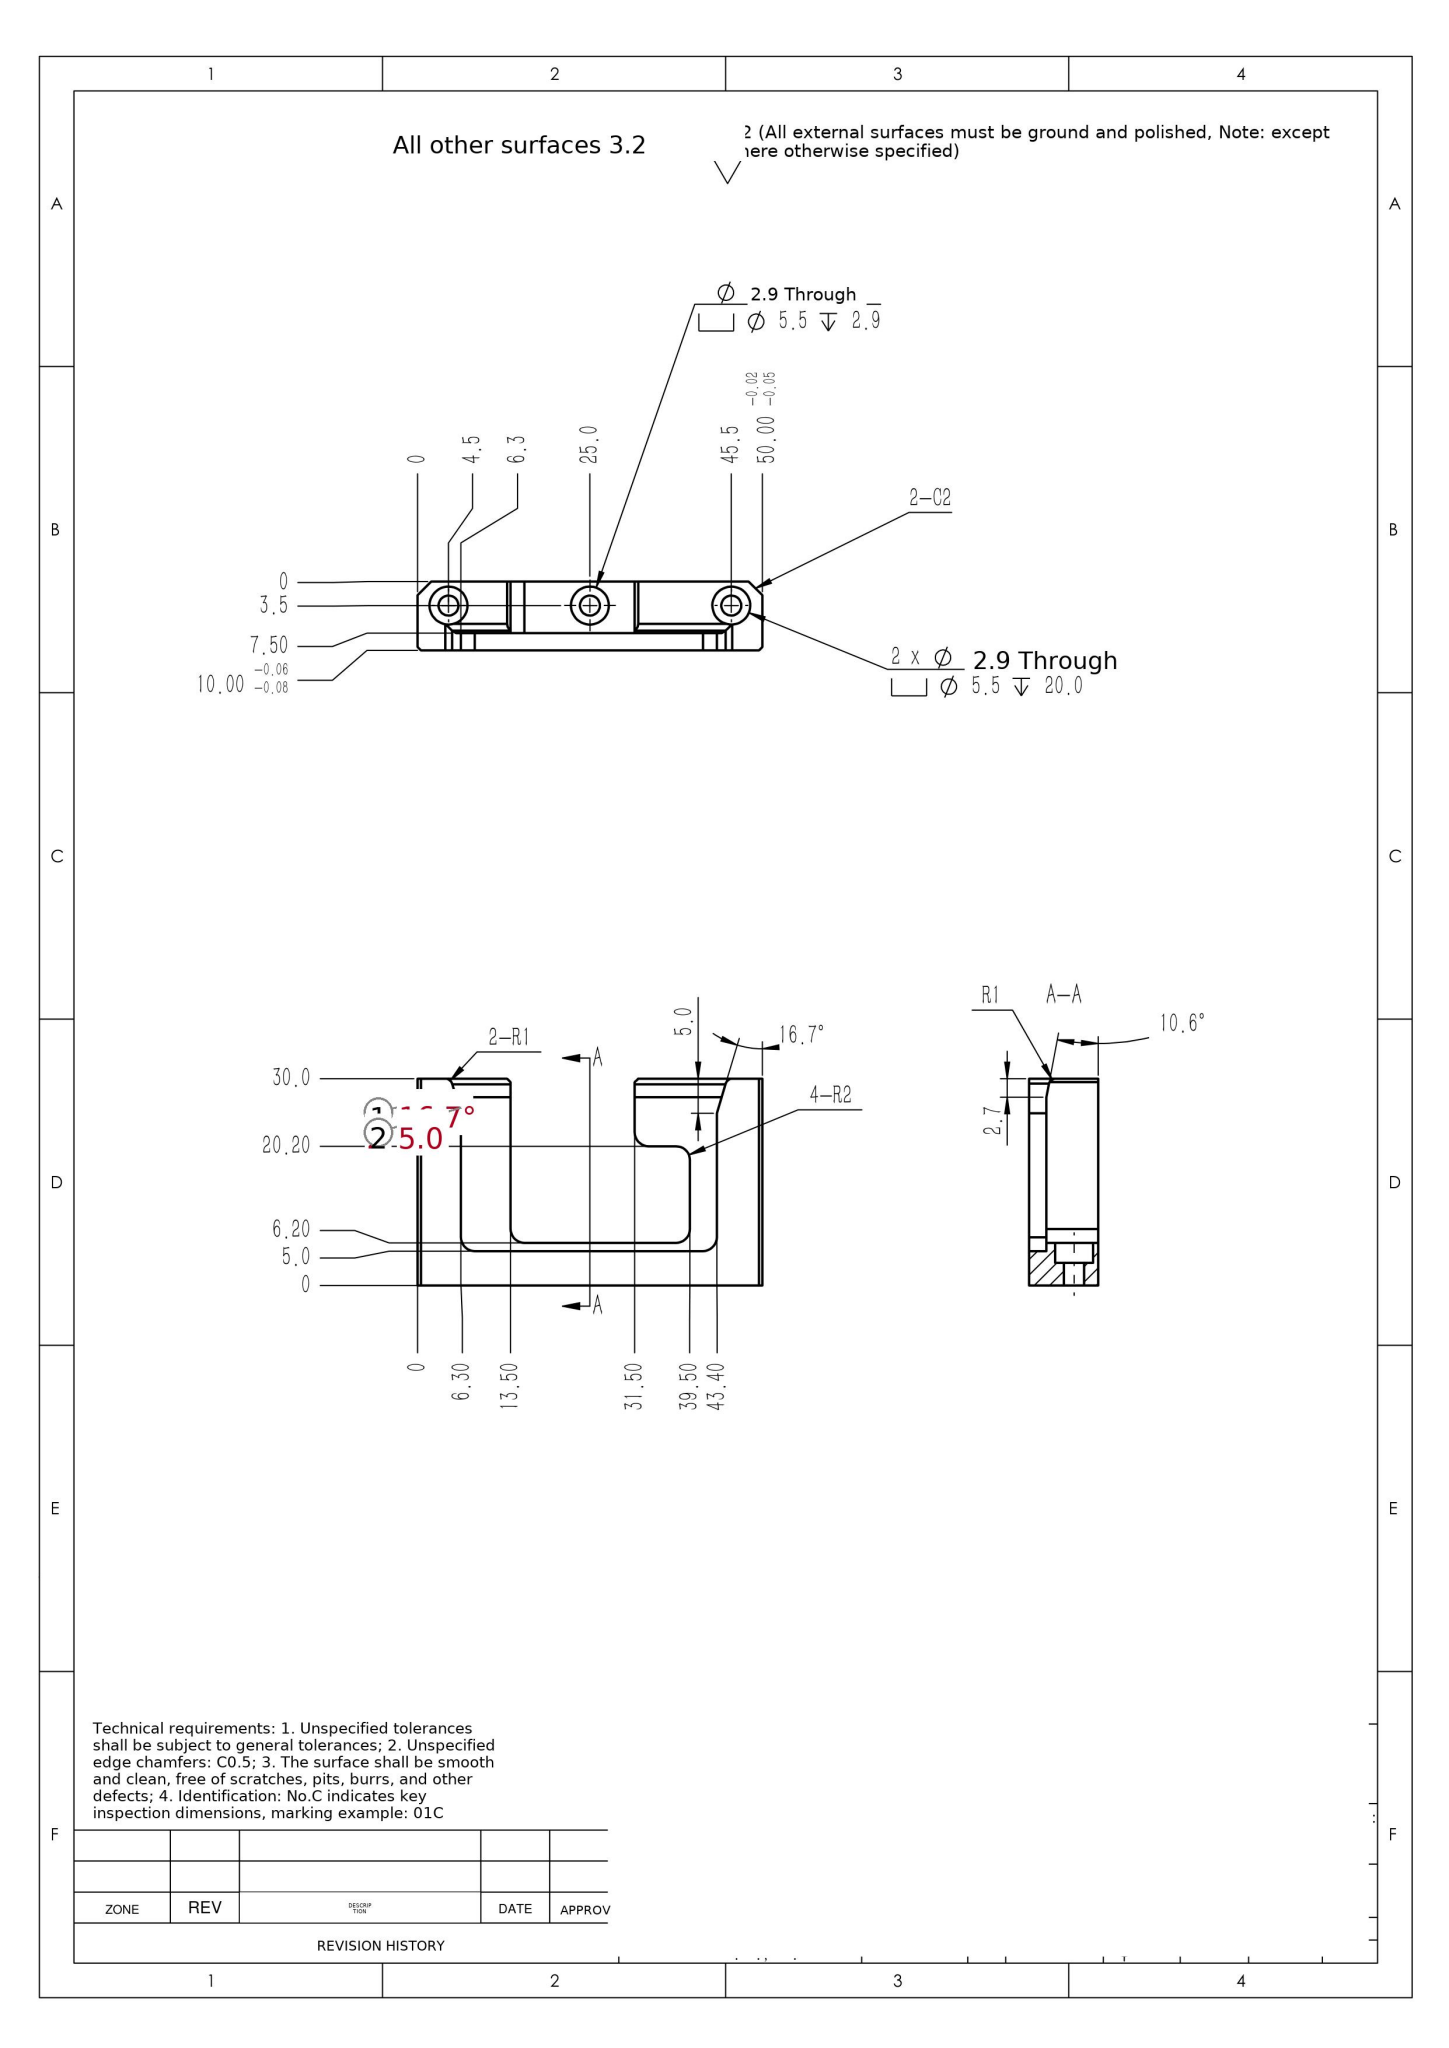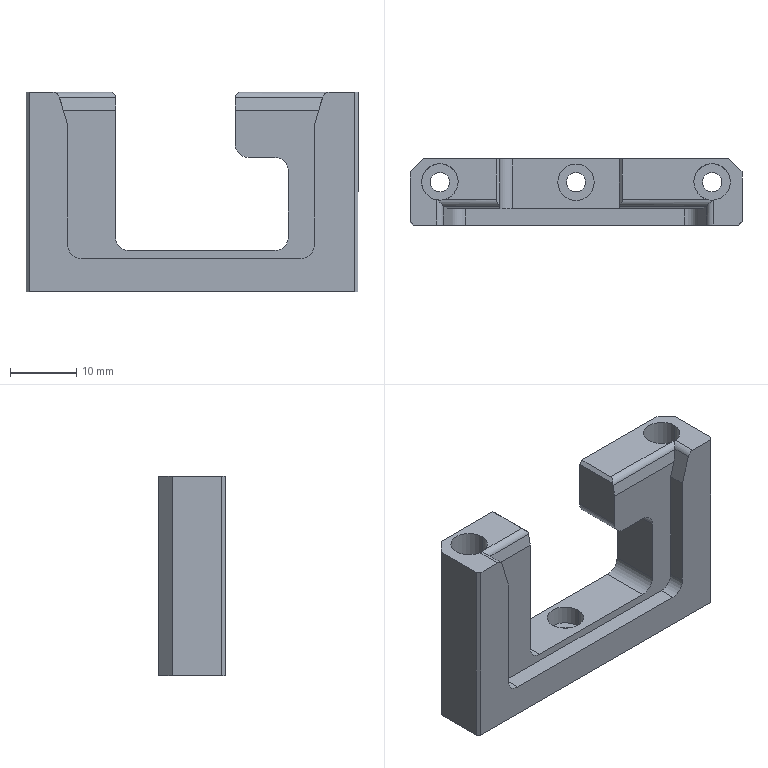Part | SolidWorks | mm | 1 solid | 51 faces | box 50 x 10 x 30 mm | volume 7306 mm3 | plane 29 | cylinder 22 | commonest cylinder face diameters 5.5 x6 2.9 x6 4 x6 2 x4